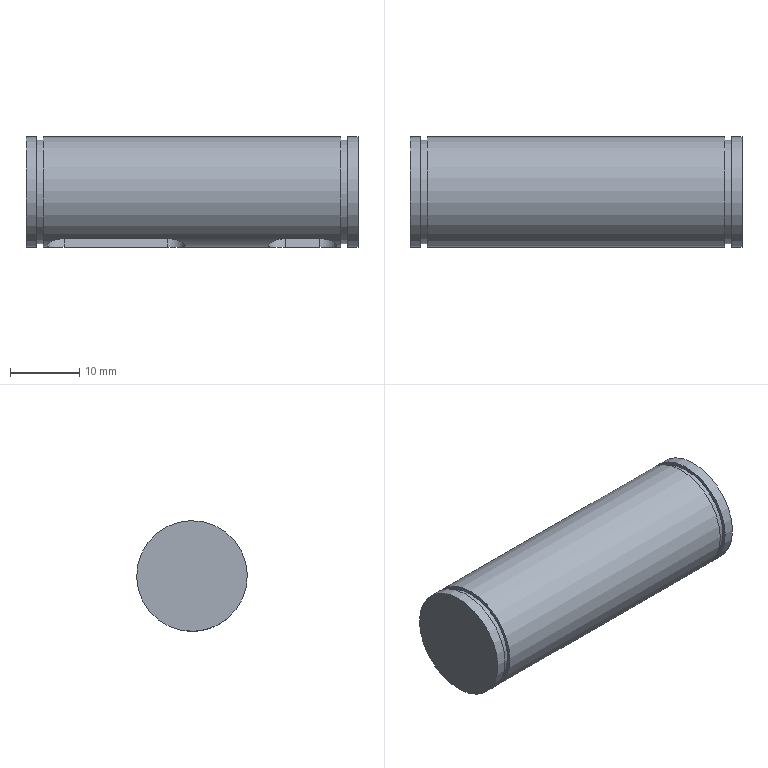Component | NX | SHAFT | 1 solid | 25 faces | volume 9272 mm3 | plane 12 | cylinder 11 | torus 2 | commonest cylinder face diameters 5 x4 16 x3 15 x2 0.4 x2